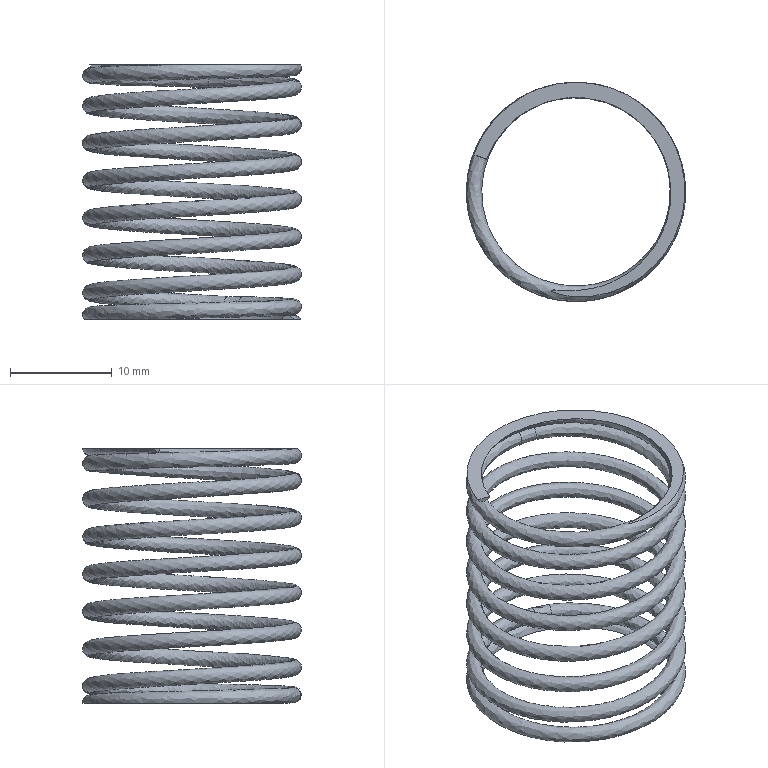Component | NX | SPRING_CYLINDER_COMPRESSION_1 | 1 solid | 9 faces | volume 898 mm3 | spline 5 | plane 4